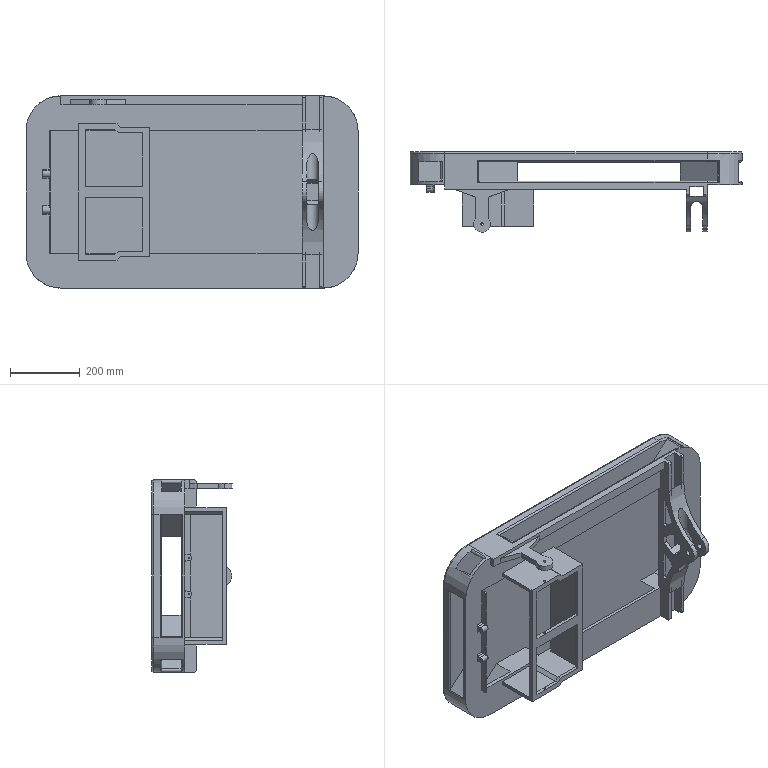Component | SolidWorks | Tray-2 | 1 solid | 224 faces | volume 22646353 mm3 | plane 117 | cylinder 93 | torus 14 | commonest cylinder face diameters 10 x55 8 x13 4 x4 16.618 x4 200 x4 48 x3 70 x2 40 x2